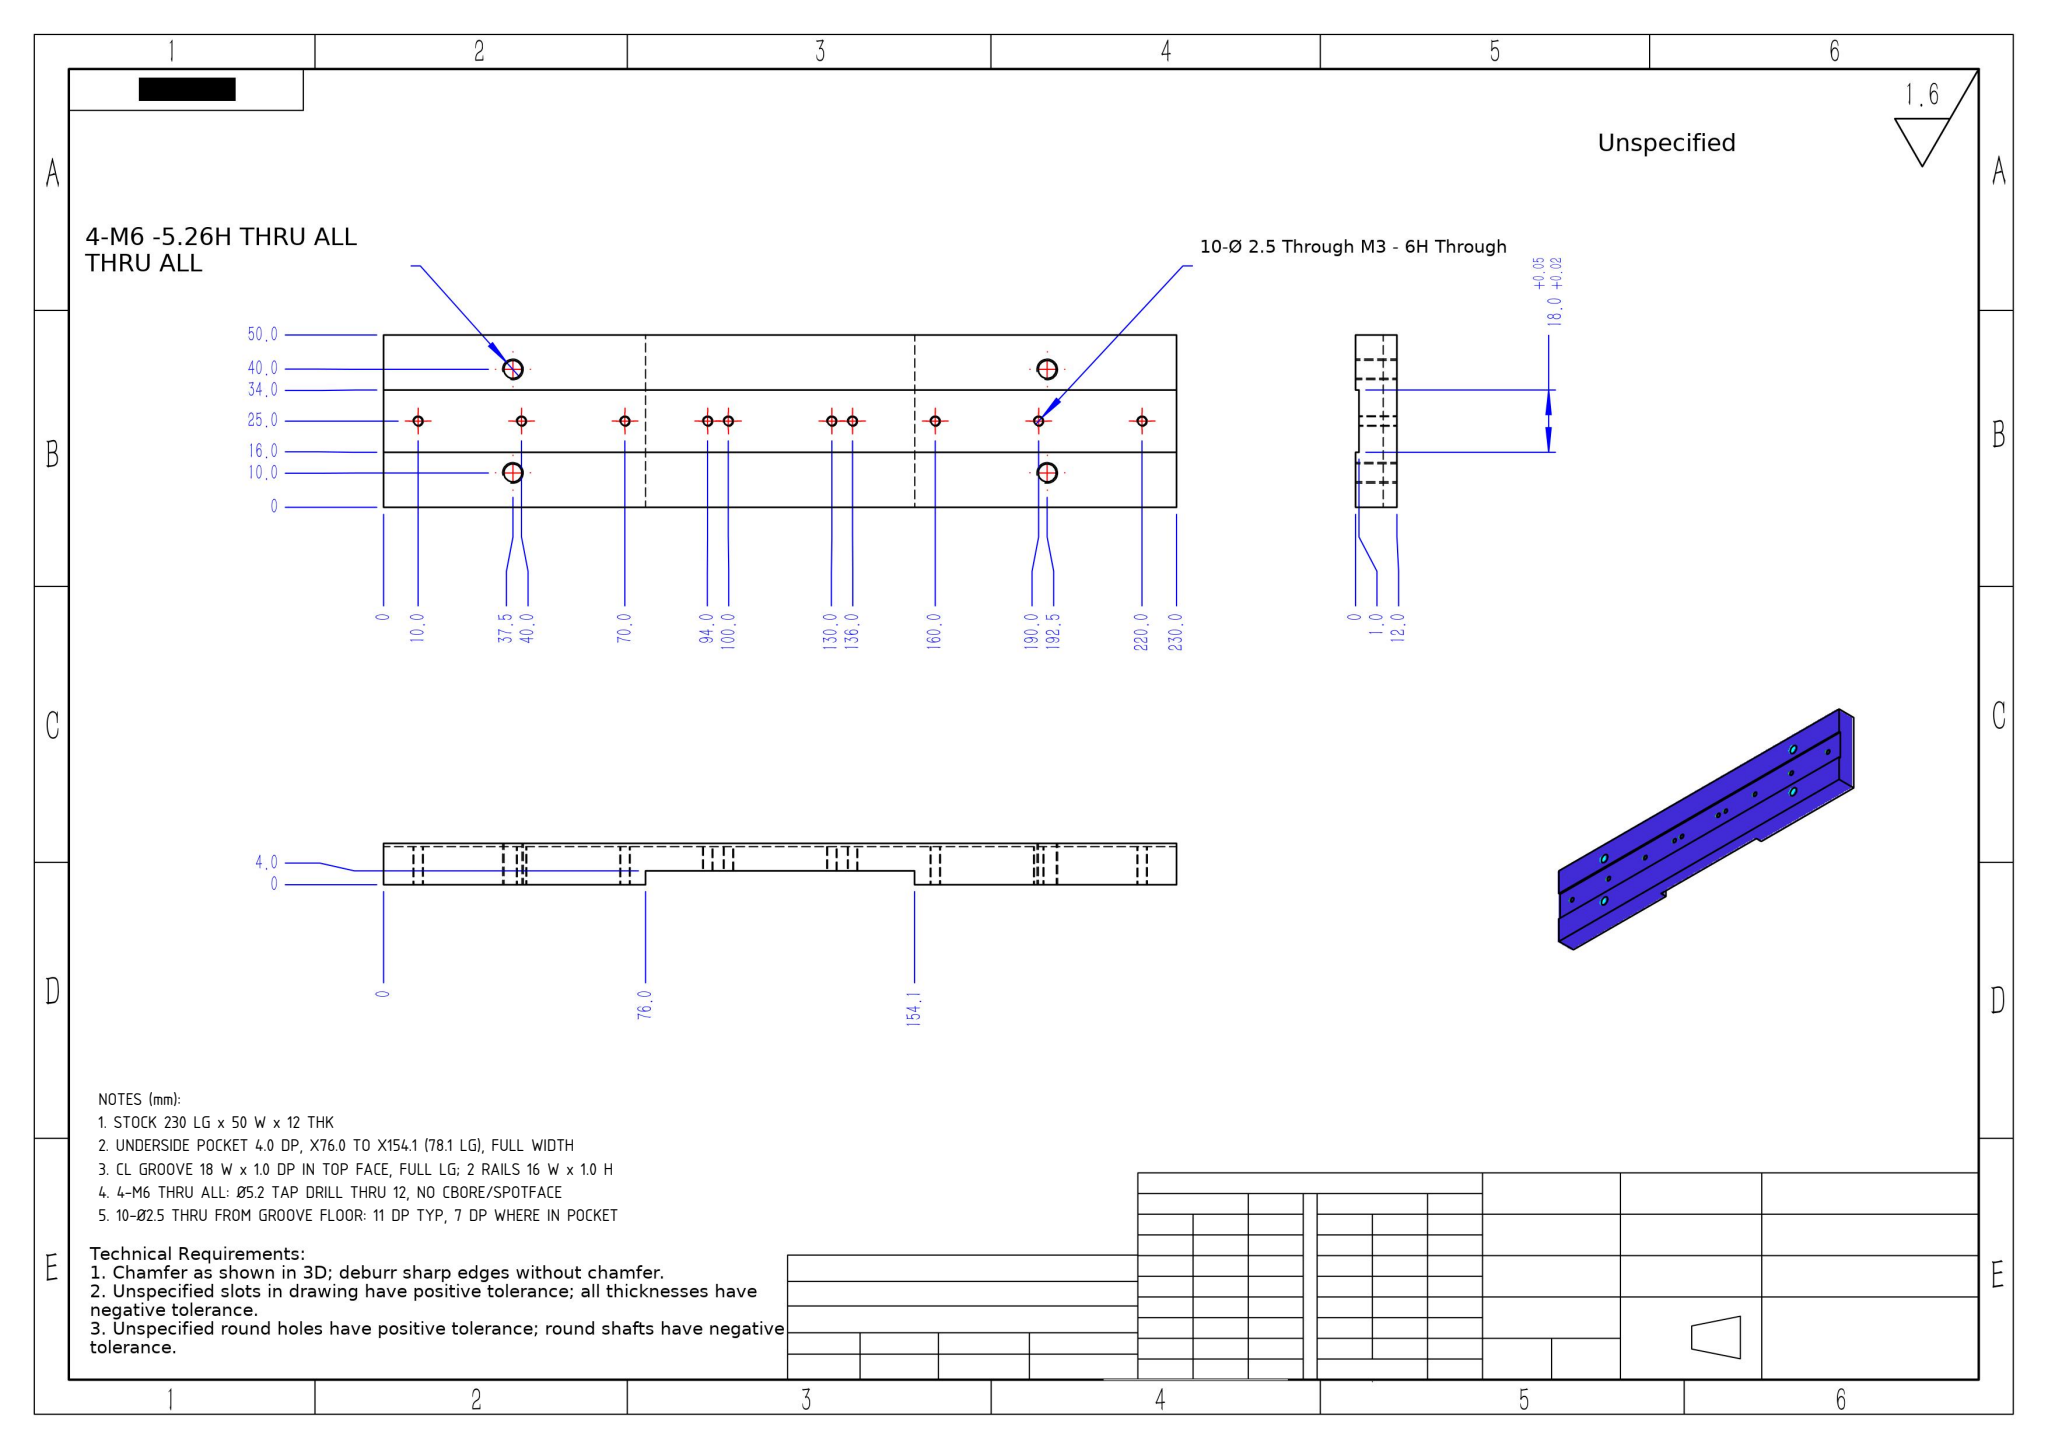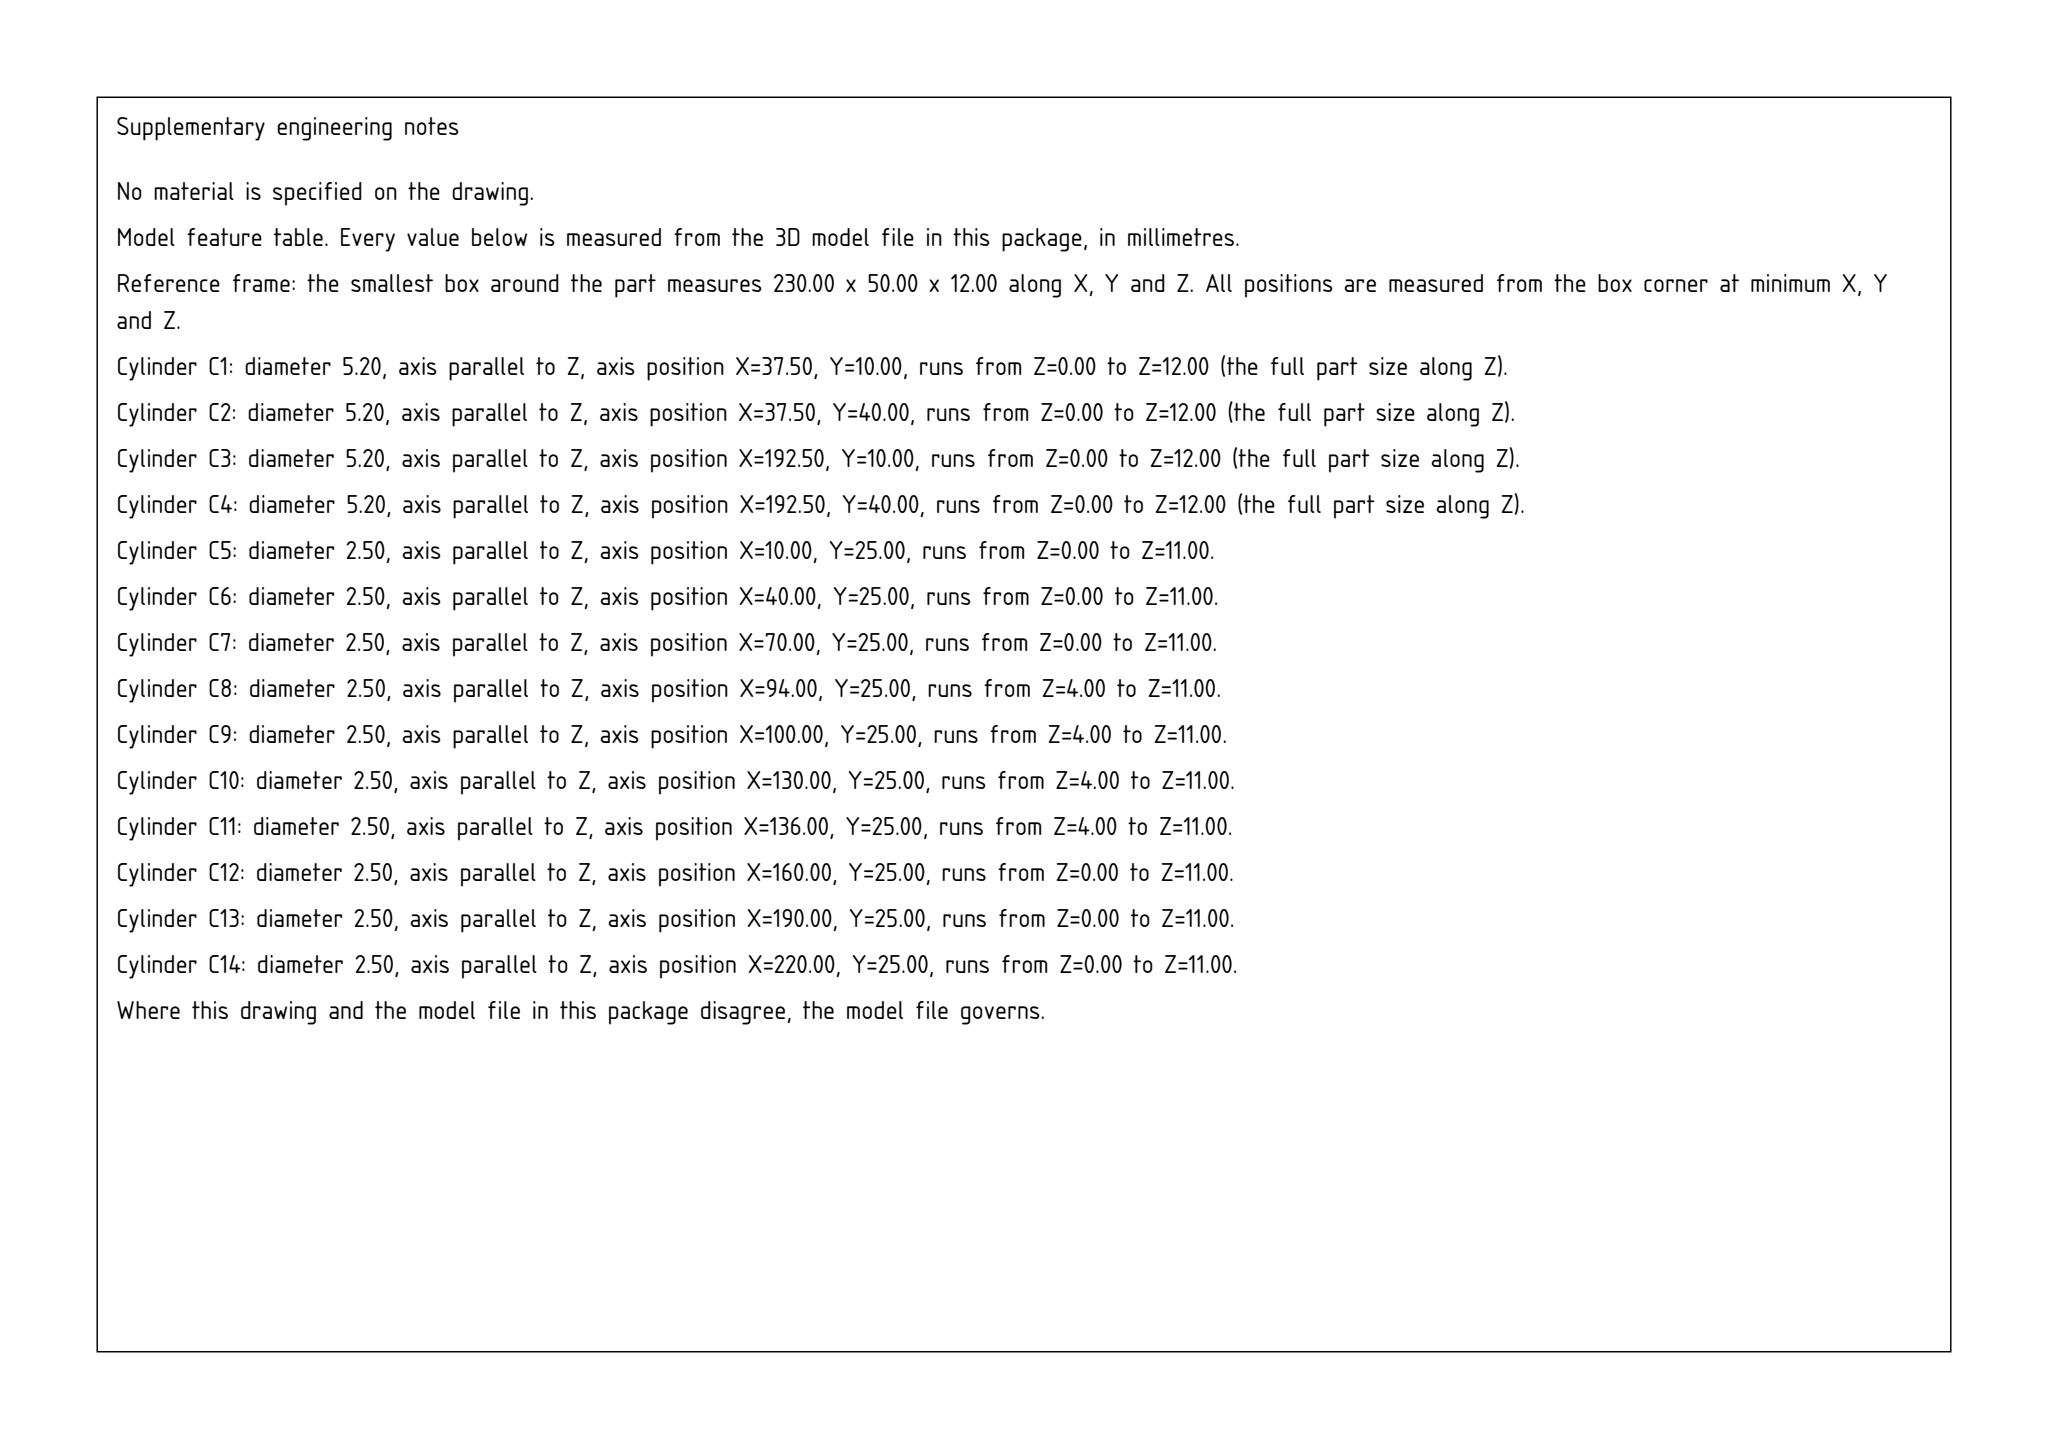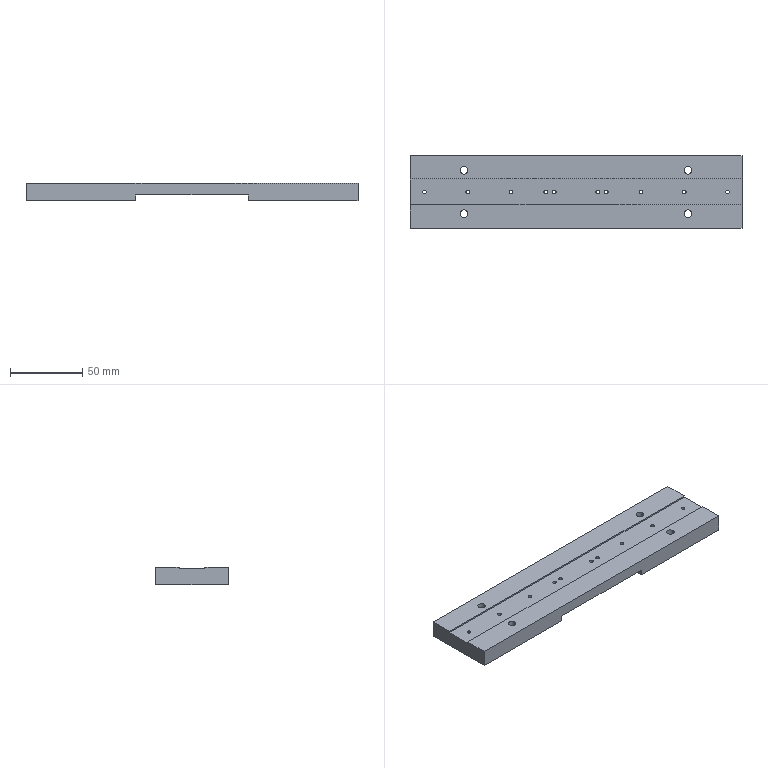Part | SolidWorks | mm | 1 solid | 42 faces | box 230 x 50 x 12 mm | volume 116759 mm3 | cylinder 28 | plane 14 | commonest cylinder face diameters 2.5 x20 5.2 x8
Drawing notes:
STOCK 230 LG x 50 W x 12 THK | from the solid: bbox_xyz 230.0 x 50.0 x 12.0
UNDERSIDE POCKET 4.0 DP, X76.0 TO X154.1 (78.1 LG), FULL WIDTH | from the solid: x-planes 75.95 & 154.05 (78.1 apart); z-planes 0.0 outer bottoms, 4.0 pocket floor
CL GROOVE 18 W x 1.0 DP IN TOP FACE, FULL LG; 2 RAILS 16 W x 1.0 H | from the solid: y-planes 0/16/34/50 = 16-18-16 bands; z-planes 11.0 groove floor vs 12.0 top faces
4-M6 THRU ALL: Ø5.2 TAP DRILL THRU 12, NO CBORE/SPOTFACE | from the solid: 4x Ø5.2 z-cyl len 12.0 at (37.5,10),(37.5,40),(192.5,10),(192.5,40)
10-Ø2.5 THRU FROM GROOVE FLOOR: 11 DP TYP, 7 DP WHERE IN POCKET | from the solid: Ø2.5 z-cyls len 11.0 at x=10,40,70,160,190,220; len 7.0 at x=94,100,130,136
build123d program:
from build123d import *

# Parameters (mm, degrees)
SKETCH1_W           = 230
SKETCH1_H           = 50
BOSS_EXTRUDE1_DEPTH = 6
SKETCH10_W          = 230
SKETCH10_H          = 18
CUT_EXTRUDE1_DEPTH  = 1
SKETCH11_W          = 78.1
SKETCH11_H          = 50
CUT_EXTRUDE2_DEPTH  = 4
M6_TAPPED_HOLE1_D   = 5.2
M3_TAPPED_HOLE1_D   = 2.5
M3_TAPPED_HOLE2_D   = 2.5


with BuildPart() as part:
    # Sketch1 → Boss-Extrude1 (new, symmetric)
    with BuildSketch(Plane.XY):
        Rectangle(SKETCH1_W, SKETCH1_H)
    extrude(amount=BOSS_EXTRUDE1_DEPTH, both=True)

    # Sketch10 → Cut-Extrude1 (cut)
    with BuildSketch(Plane.XY.offset(6)):
        Rectangle(SKETCH10_W, SKETCH10_H)
    extrude(amount=-CUT_EXTRUDE1_DEPTH, mode=Mode.SUBTRACT)

    # Sketch11 → Cut-Extrude2 (cut)
    with BuildSketch(Plane(origin=(0, 0, -6), x_dir=(-1, 0, 0), z_dir=(0, 0, -1))):
        Rectangle(SKETCH11_W, SKETCH11_H)
    extrude(amount=-CUT_EXTRUDE2_DEPTH, mode=Mode.SUBTRACT)

    # M6 Tapped Hole1 (through all)
    with Locations(Plane(origin=(0, 0, -6), x_dir=(-1, 0, 0), z_dir=(0, 0, -1))):
        with Locations((-77.5, 15), (-77.5, -15), (77.5, -15), (77.5, 15)):
            Hole(M6_TAPPED_HOLE1_D / 2)

    # M3 Tapped Hole1 (through all)
    with Locations(Plane.XY.offset(6)):
        with Locations((105, 0), (-105, 0), (-75, 0), (-45, 0), (-15, 0), (15, 0), (45, 0), (75, 0)):
            Hole(M3_TAPPED_HOLE1_D / 2)

    # M3 Tapped Hole2 (through all)
    with Locations(Plane(origin=(0, 0, -6), x_dir=(-1, 0, 0), z_dir=(0, 0, -1))):
        with Locations((-21, 0), (21, 0)):
            Hole(M3_TAPPED_HOLE2_D / 2)


solid = part.part